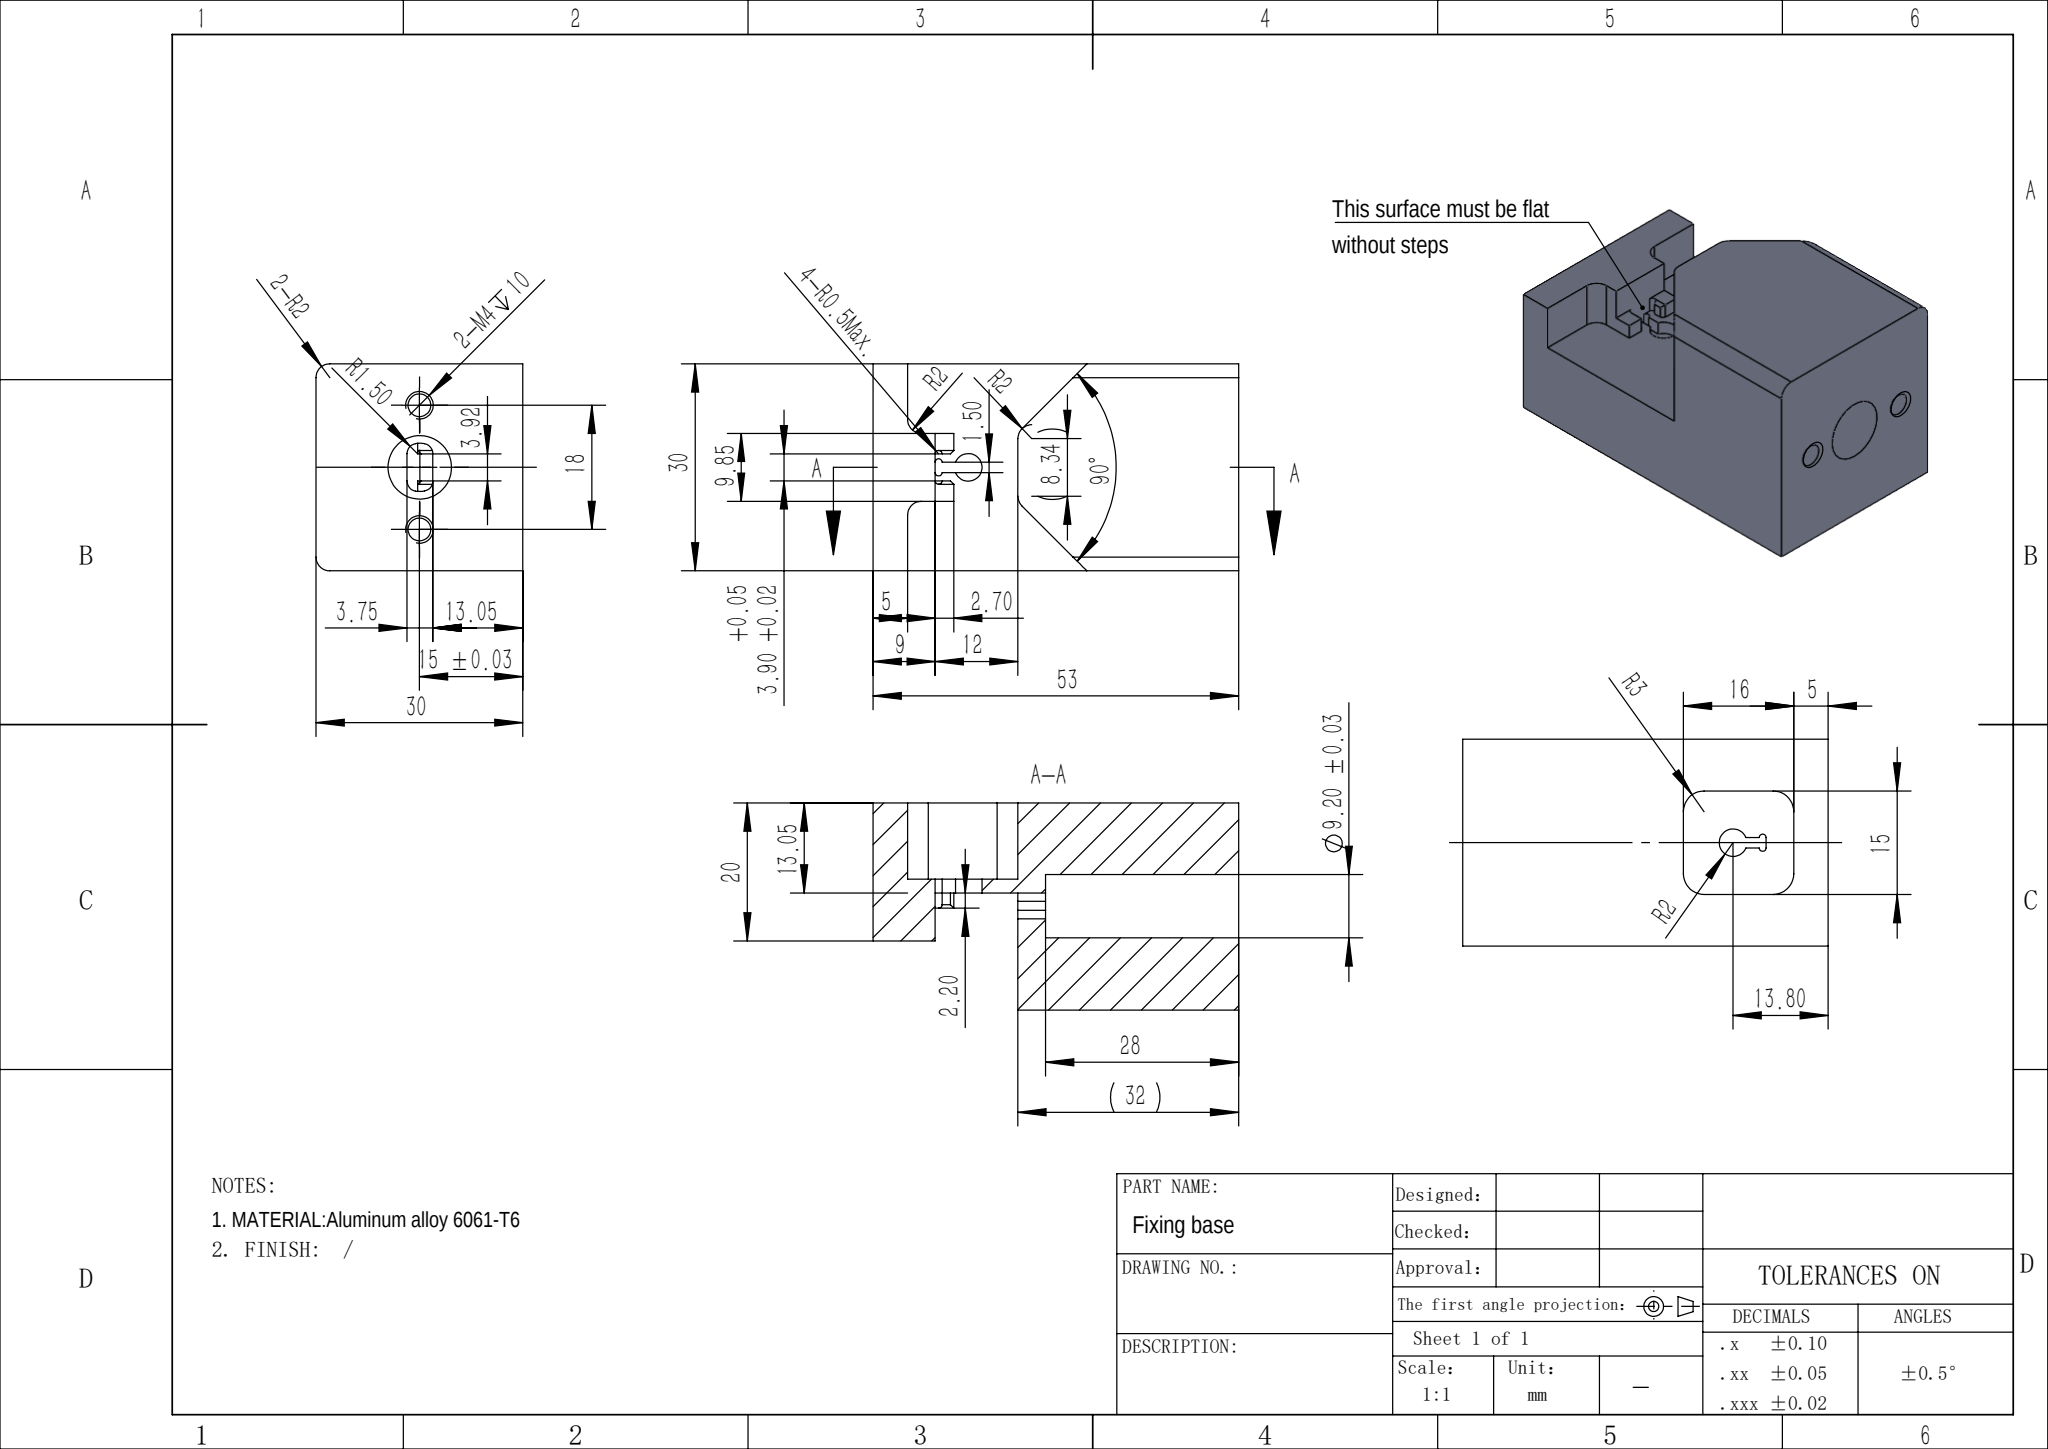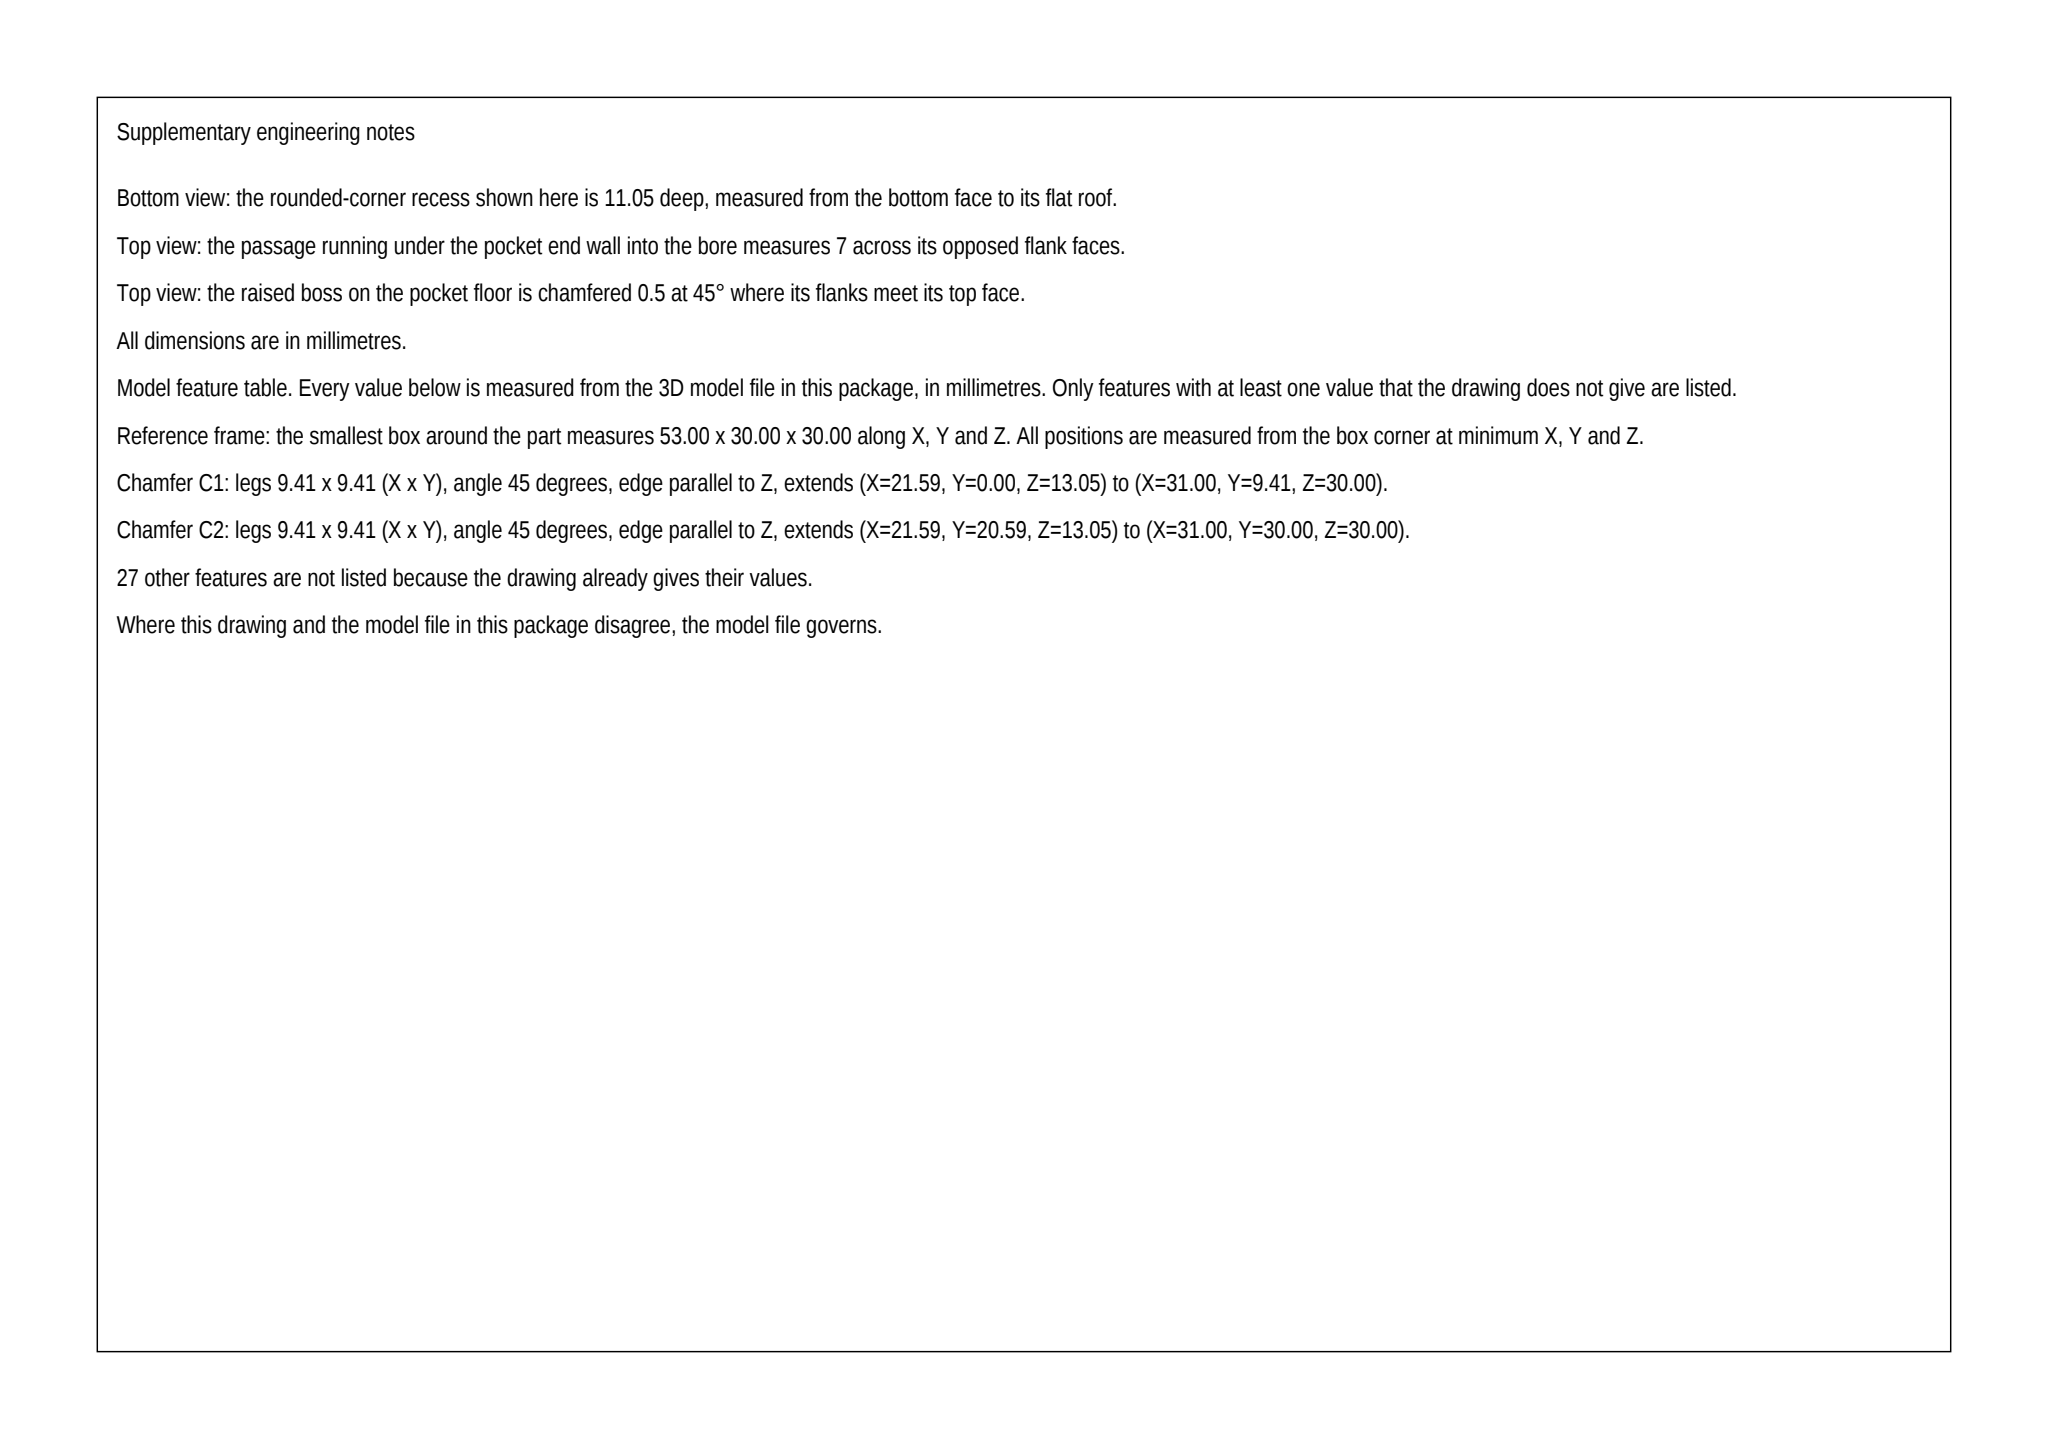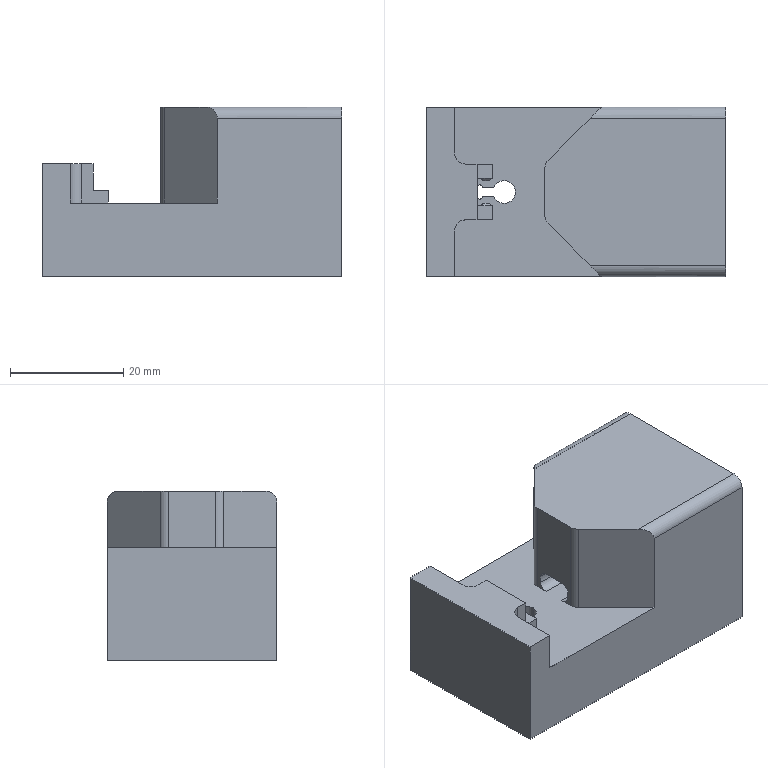Part | SolidWorks | mm | material Aluminum alloy 6061-T6 | 1 solid | 67 faces | box 53 x 30 x 30 mm | volume 31910 mm3 | plane 35 | cylinder 28 | cone 4 | commonest cylinder face diameters 4 x8 3.3 x4 1 x4 3 x4 6 x4 9.2 x2 7 x2